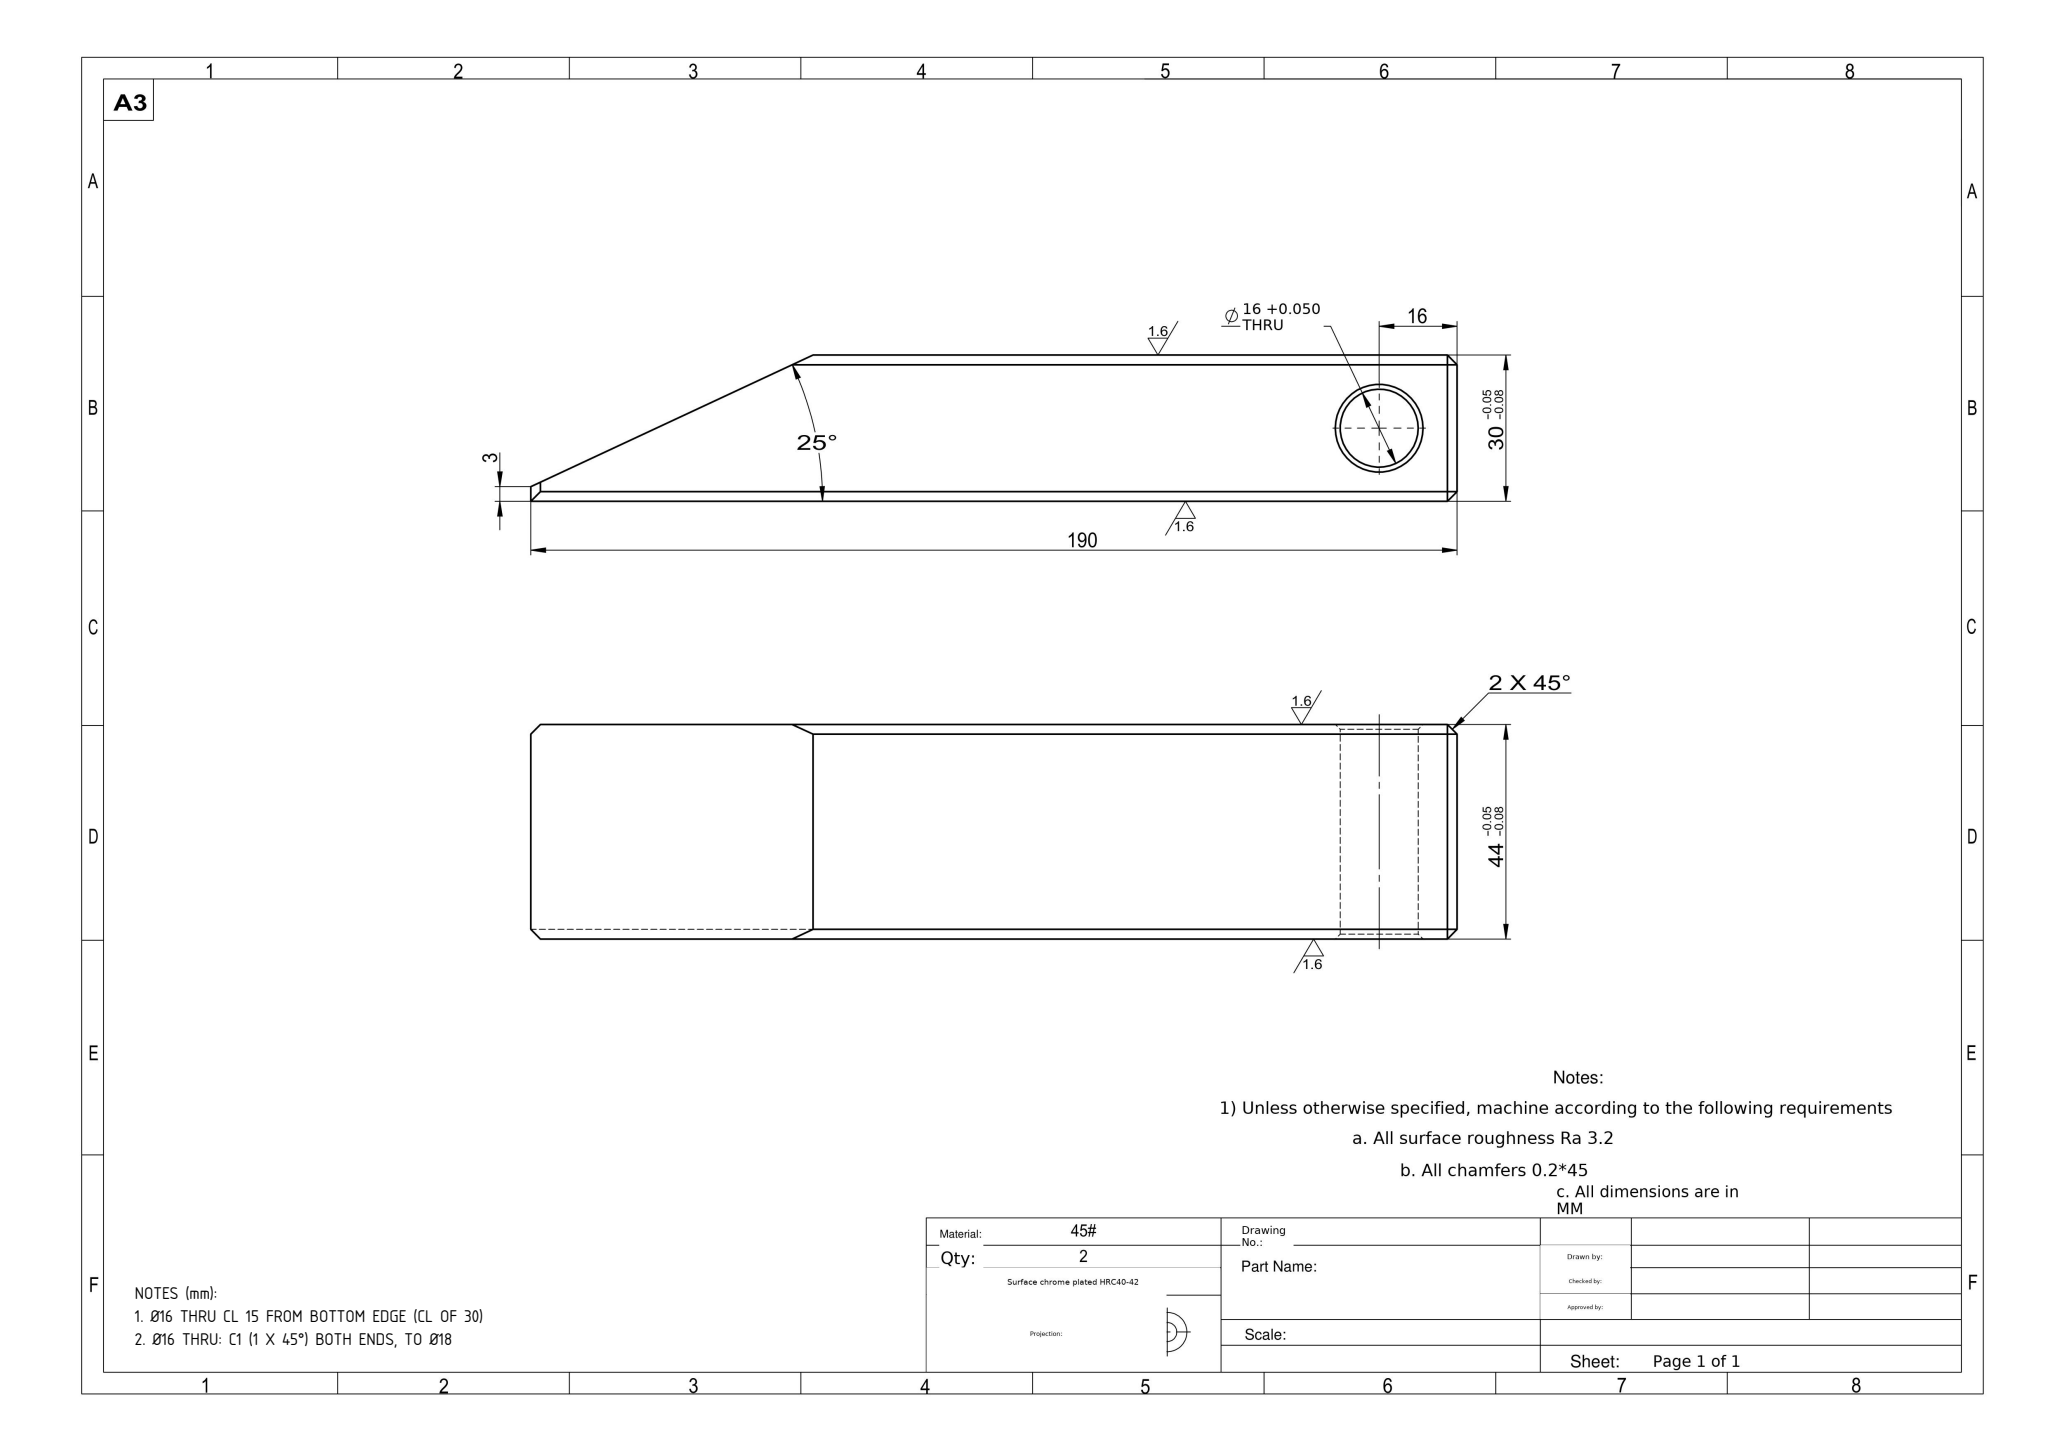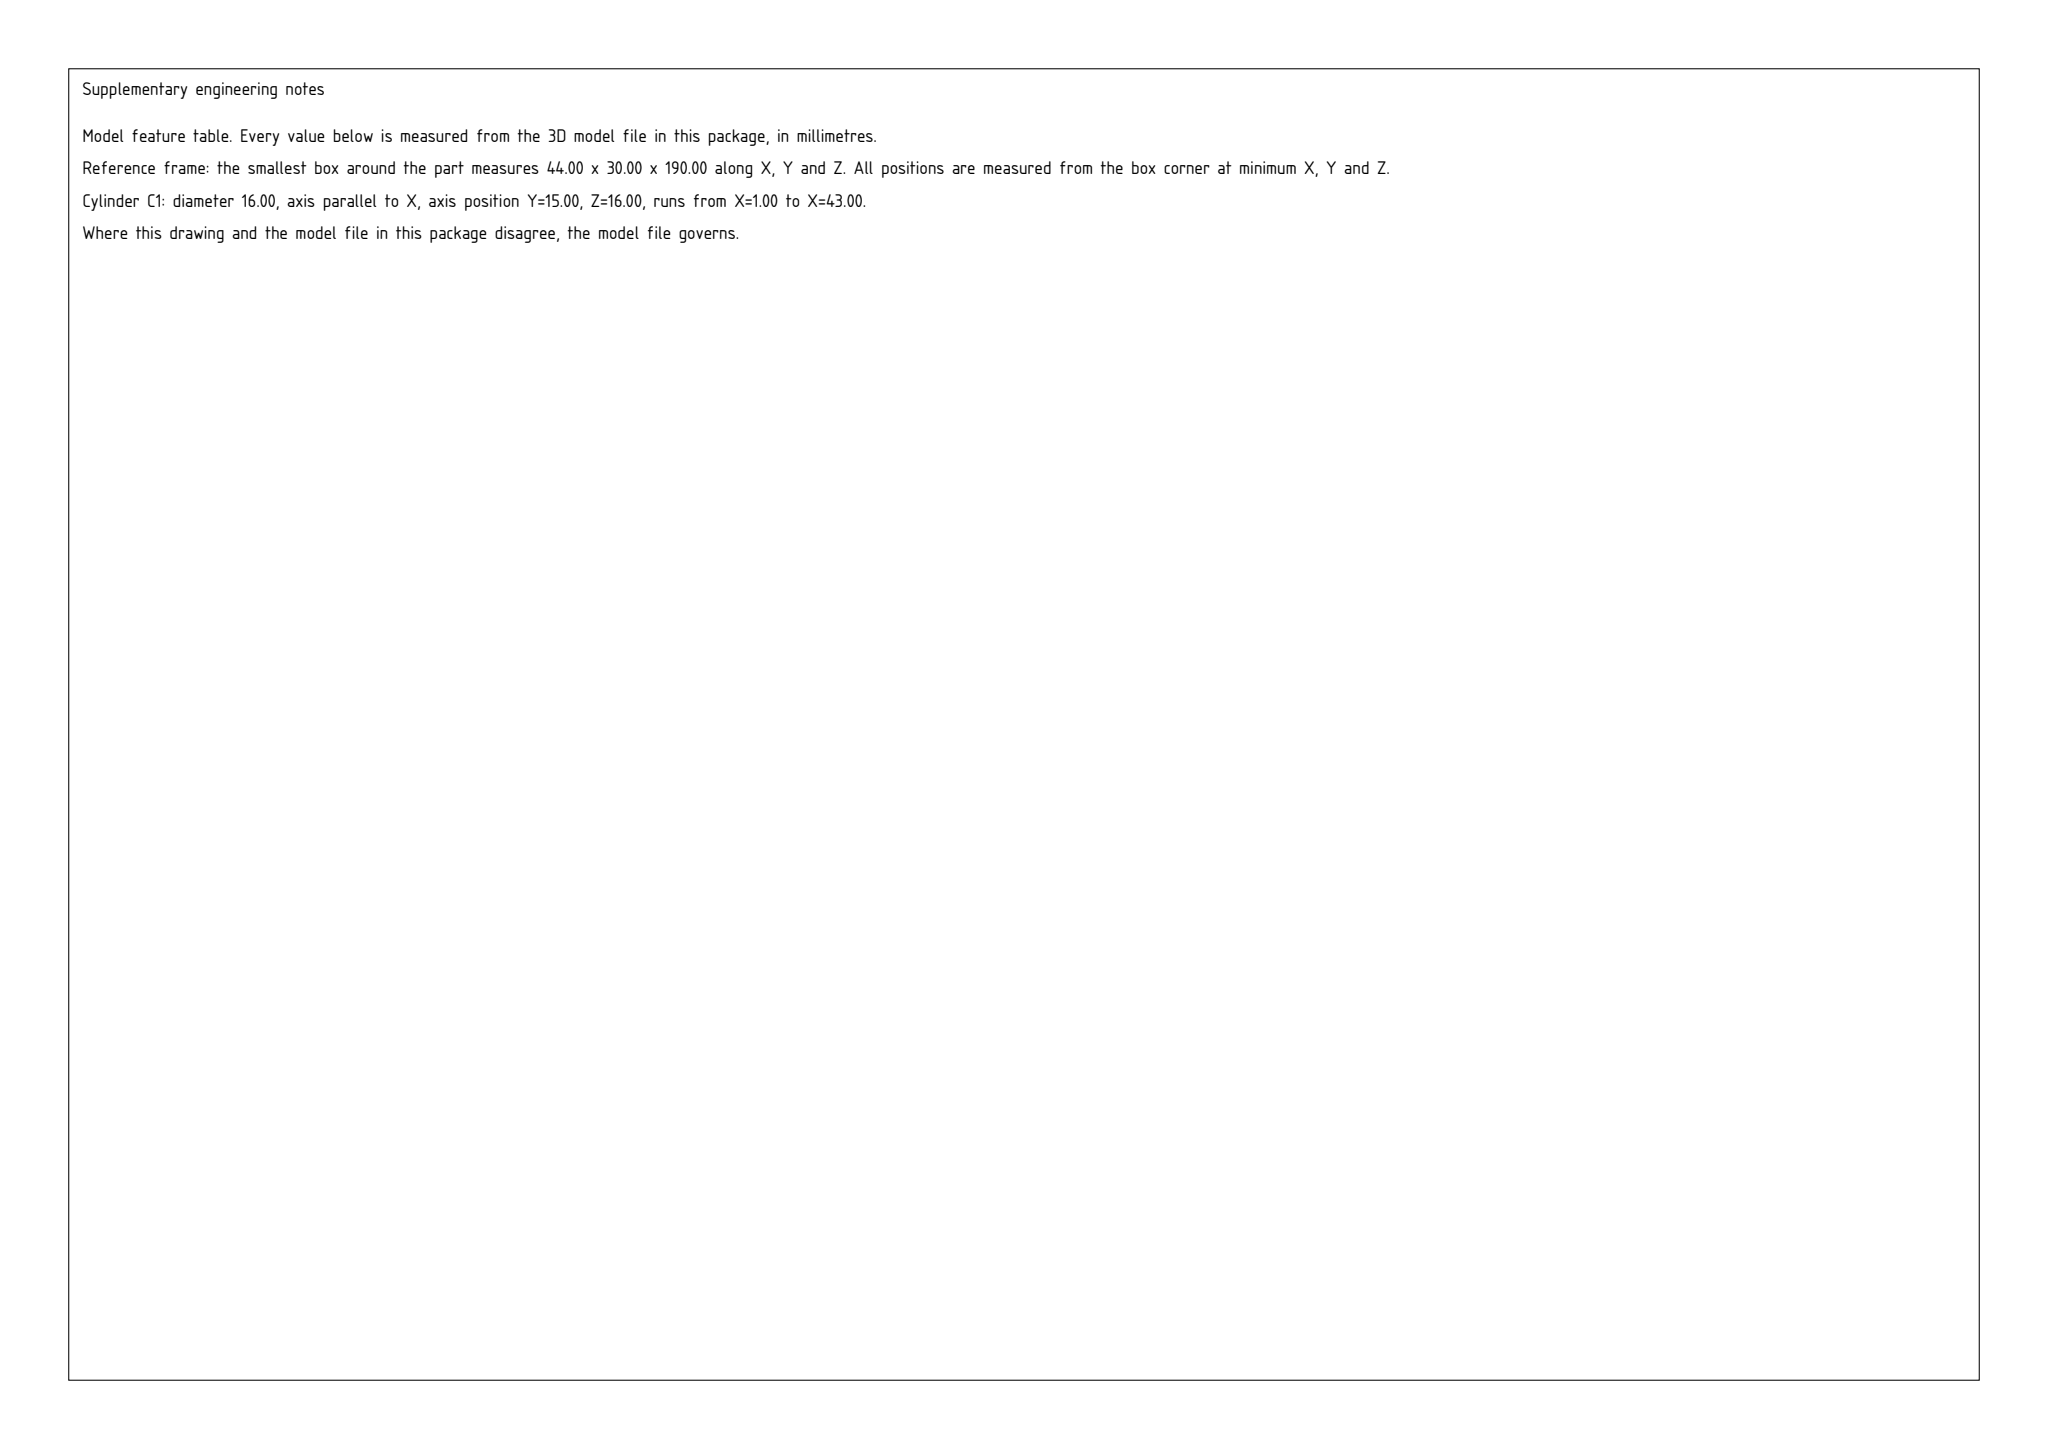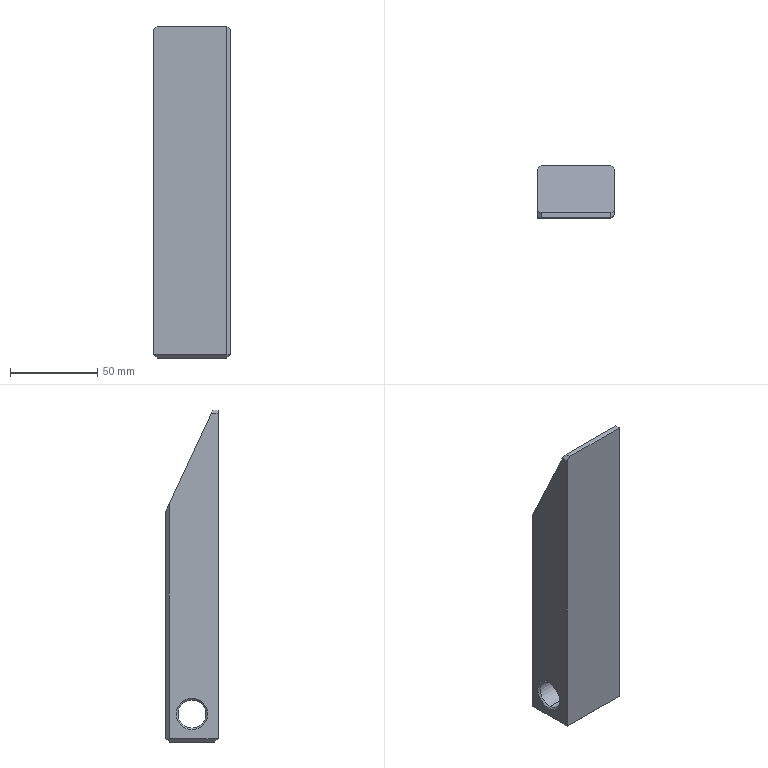Part | SolidWorks | mm | 1 solid | 25 faces | box 44 x 30 x 190 mm | volume 206305 mm3 | plane 19 | cone 4 | cylinder 2 | commonest cylinder face diameters 16 x2
Drawing notes:
Ø16 THRU CL 15 FROM BOTTOM EDGE (CL OF 30) | from the solid: cylinder dia 16, axis x, y=15 of 30 bbox height
Ø16 THRU: C1 (1 X 45°) BOTH ENDS, TO Ø18 | from the solid: cyl length 42 in 44 wide block; cones 90 incl, ref dia 18 at both ends
build123d program:
from build123d import *

# Parameters (mm, degrees)
BOSS_EXTRUDE1_DEPTH        = 22
F_16_0_16_DIAMETER_HOLE1_D = 16
CHAMFER1_SIZE              = 2
CHAMFER2_SIZE              = 1


with BuildPart() as part:
    # Sketch1 → Boss-Extrude1 (new, symmetric)
    with BuildSketch(Plane(origin=(0, 0, 0), x_dir=(0, 0, -1), z_dir=(1, 0, 0))):
        Polygon((-95, 0), (95, 0), (95, 30), (-37.098, 30), (-95, 3), align=None)
    extrude(amount=BOSS_EXTRUDE1_DEPTH, both=True)

    # 16.0 _16_ Diameter Hole1 (through all)
    with Locations(Plane(origin=(22, 0, 0), x_dir=(0, 0, -1), z_dir=(1, 0, 0))):
        with Locations((79, 15)):
            Hole(F_16_0_16_DIAMETER_HOLE1_D / 2)

    # Chamfer1
    chamfer1_edges = [part.edges().sort_by_distance(p)[0] for p in [
        (22, 15, -95),
        (22, 30, -28.951),
        (22, 1.5, 95),
        (-22, 30, -28.951),
        (-22, 15, -95),
        (-22, 1.5, 95),
        (22, 0, 0),
        (0, 30, -95),
        (0, 0, -95),
    ]]
    chamfer(chamfer1_edges, length=CHAMFER1_SIZE)

    # Chamfer2
    chamfer2_edges = [part.edges().sort_by_distance(p)[0] for p in [
        (22, 15, -87),
        (-22, 15, -87),
    ]]
    chamfer(chamfer2_edges, length=CHAMFER2_SIZE)


solid = part.part
STEP:
#1=CARTESIAN_POINT('',(-21.,15.,-87.));
#2=VERTEX_POINT('',#1);
#3=CARTESIAN_POINT('',(-21.,15.,-71.));
#4=VERTEX_POINT('',#3);
#5=CARTESIAN_POINT('',(-21.,15.,-79.));
#6=DIRECTION('',(-1.,0.,0.));
#7=DIRECTION('',(0.,0.,-1.));
#8=AXIS2_PLACEMENT_3D('',#5,#6,#7);
#9=CIRCLE('',#8,8.);
#10=EDGE_CURVE('',#2,#4,#9,.T.);
#11=ORIENTED_EDGE('',*,*,#10,.F.);
#12=CARTESIAN_POINT('',(-22.,15.,-88.));
#13=VERTEX_POINT('',#12);
#14=CARTESIAN_POINT('',(-22.,15.,-88.));
#15=DIRECTION('',(-0.7071,0.,-0.7071));
#16=VECTOR('',#15,1000.);
#17=LINE('',#14,#16);
#18=EDGE_CURVE('',#2,#13,#17,.T.);
#19=ORIENTED_EDGE('',*,*,#18,.T.);
#20=CARTESIAN_POINT('',(-22.,15.,-70.));
#21=VERTEX_POINT('',#20);
#22=CARTESIAN_POINT('',(-22.,15.,-79.));
#23=DIRECTION('',(1.,0.,0.));
#24=DIRECTION('',(0.,0.,-1.));
#25=AXIS2_PLACEMENT_3D('',#22,#23,#24);
#26=CIRCLE('',#25,9.);
#27=EDGE_CURVE('',#21,#13,#26,.T.);
#28=ORIENTED_EDGE('',*,*,#27,.F.);
#29=CARTESIAN_POINT('',(-22.,15.,-70.));
#30=DIRECTION('',(-0.7071,0.,0.7071));
#31=VECTOR('',#30,1000.);
#32=LINE('',#29,#31);
#33=EDGE_CURVE('',#4,#21,#32,.T.);
#34=ORIENTED_EDGE('',*,*,#33,.F.);
#35=EDGE_LOOP('',(#11,#19,#28,#34));
#36=FACE_OUTER_BOUND('',#35,.T.);
#37=CARTESIAN_POINT('',(-22.,15.,-79.));
#38=DIRECTION('',(-1.,0.,0.));
#39=DIRECTION('',(0.,0.,1.));
#40=AXIS2_PLACEMENT_3D('',#37,#38,#39);
#41=CONICAL_SURFACE('',#40,9.,0.7854);
#42=ADVANCED_FACE('',(#36),#41,.F.);
#43=CARTESIAN_POINT('',(21.,15.,-71.));
#44=VERTEX_POINT('',#43);
#45=CARTESIAN_POINT('',(21.,15.,-87.));
#46=VERTEX_POINT('',#45);
#47=CARTESIAN_POINT('',(21.,15.,-79.));
#48=DIRECTION('',(1.,0.,0.));
#49=DIRECTION('',(0.,0.,-1.));
#50=AXIS2_PLACEMENT_3D('',#47,#48,#49);
#51=CIRCLE('',#50,8.);
#52=EDGE_CURVE('',#44,#46,#51,.T.);
#53=ORIENTED_EDGE('',*,*,#52,.F.);
#54=CARTESIAN_POINT('',(22.,15.,-70.));
#55=VERTEX_POINT('',#54);
#56=CARTESIAN_POINT('',(21.,15.,-71.));
#57=DIRECTION('',(0.7071,0.,0.7071));
#58=VECTOR('',#57,1000.);
#59=LINE('',#56,#58);
#60=EDGE_CURVE('',#44,#55,#59,.T.);
#61=ORIENTED_EDGE('',*,*,#60,.T.);
#62=CARTESIAN_POINT('',(22.,15.,-88.));
#63=VERTEX_POINT('',#62);
#64=CARTESIAN_POINT('',(22.,15.,-79.));
#65=DIRECTION('',(-1.,0.,0.));
#66=DIRECTION('',(0.,0.,-1.));
#67=AXIS2_PLACEMENT_3D('',#64,#65,#66);
#68=CIRCLE('',#67,9.);
#69=EDGE_CURVE('',#63,#55,#68,.T.);
#70=ORIENTED_EDGE('',*,*,#69,.F.);
#71=CARTESIAN_POINT('',(21.,15.,-87.));
#72=DIRECTION('',(0.7071,0.,-0.7071));
#73=VECTOR('',#72,1000.);
#74=LINE('',#71,#73);
#75=EDGE_CURVE('',#46,#63,#74,.T.);
#76=ORIENTED_EDGE('',*,*,#75,.F.);
#77=EDGE_LOOP('',(#53,#61,#70,#76));
#78=FACE_OUTER_BOUND('',#77,.T.);
#79=CARTESIAN_POINT('',(21.,15.,-79.));
#80=DIRECTION('',(1.,0.,0.));
#81=DIRECTION('',(0.,0.,-1.));
#82=AXIS2_PLACEMENT_3D('',#79,#80,#81);
#83=CONICAL_SURFACE('',#82,8.,0.7854);
#84=ADVANCED_FACE('',(#78),#83,.F.);
#85=ORIENTED_EDGE('',*,*,#10,.T.);
#86=CARTESIAN_POINT('',(22.,15.,-71.));
#87=DIRECTION('',(1.,0.,0.));
#88=VECTOR('',#87,1000.);
#89=LINE('',#86,#88);
#90=EDGE_CURVE('',#4,#44,#89,.T.);
#91=ORIENTED_EDGE('',*,*,#90,.T.);
#92=ORIENTED_EDGE('',*,*,#52,.T.);
#93=CARTESIAN_POINT('',(22.,15.,-87.));
#94=DIRECTION('',(1.,0.,0.));
#95=VECTOR('',#94,1000.);
#96=LINE('',#93,#95);
#97=EDGE_CURVE('',#2,#46,#96,.T.);
#98=ORIENTED_EDGE('',*,*,#97,.F.);
#99=EDGE_LOOP('',(#85,#91,#92,#98));
#100=FACE_OUTER_BOUND('',#99,.T.);
#101=CARTESIAN_POINT('',(22.,15.,-79.));
#102=DIRECTION('',(1.,0.,0.));
#103=DIRECTION('',(0.,0.,-1.));
#104=AXIS2_PLACEMENT_3D('',#101,#102,#103);
#105=CYLINDRICAL_SURFACE('',#104,8.);
#106=ADVANCED_FACE('',(#100),#105,.F.);
#107=CARTESIAN_POINT('',(20.,3.,95.));
#108=VERTEX_POINT('',#107);
#109=CARTESIAN_POINT('',(-20.,3.,95.));
#110=VERTEX_POINT('',#109);
#111=CARTESIAN_POINT('',(22.,3.,95.));
#112=DIRECTION('',(-1.,0.,0.));
#113=VECTOR('',#112,1000.);
#114=LINE('',#111,#113);
#115=EDGE_CURVE('',#108,#110,#114,.T.);
#116=ORIENTED_EDGE('',*,*,#115,.T.);
#117=CARTESIAN_POINT('',(-20.,0.,95.));
#118=VERTEX_POINT('',#117);
#119=CARTESIAN_POINT('',(-20.,3.,95.));
#120=DIRECTION('',(0.,-1.,0.));
#121=VECTOR('',#120,1000.);
#122=LINE('',#119,#121);
#123=EDGE_CURVE('',#110,#118,#122,.T.);
#124=ORIENTED_EDGE('',*,*,#123,.T.);
#125=CARTESIAN_POINT('',(20.,0.,95.));
#126=VERTEX_POINT('',#125);
#127=CARTESIAN_POINT('',(22.,0.,95.));
#128=DIRECTION('',(-1.,0.,0.));
#129=VECTOR('',#128,1000.);
#130=LINE('',#127,#129);
#131=EDGE_CURVE('',#126,#118,#130,.T.);
#132=ORIENTED_EDGE('',*,*,#131,.F.);
#133=CARTESIAN_POINT('',(20.,3.,95.));
#134=DIRECTION('',(0.,1.,0.));
#135=VECTOR('',#134,1000.);
#136=LINE('',#133,#135);
#137=EDGE_CURVE('',#126,#108,#136,.T.);
#138=ORIENTED_EDGE('',*,*,#137,.T.);
#139=EDGE_LOOP('',(#116,#124,#132,#138));
#140=FACE_OUTER_BOUND('',#139,.T.);
#141=CARTESIAN_POINT('',(22.,3.,95.));
#142=DIRECTION('',(0.,0.,-1.));
#143=DIRECTION('',(-1.,0.,0.));
#144=AXIS2_PLACEMENT_3D('',#141,#142,#143);
#145=PLANE('',#144);
#146=ADVANCED_FACE('',(#140),#145,.F.);
#147=ORIENTED_EDGE('',*,*,#131,.T.);
#148=CARTESIAN_POINT('',(-22.,0.,93.));
#149=VERTEX_POINT('',#148);
#150=CARTESIAN_POINT('',(-20.,0.,95.));
#151=DIRECTION('',(-0.7071,0.,-0.7071));
#152=VECTOR('',#151,1000.);
#153=LINE('',#150,#152);
#154=EDGE_CURVE('',#118,#149,#153,.T.);
#155=ORIENTED_EDGE('',*,*,#154,.T.);
#156=CARTESIAN_POINT('',(-22.,0.,-93.));
#157=VERTEX_POINT('',#156);
#158=CARTESIAN_POINT('',(-22.,0.,95.));
#159=DIRECTION('',(0.,0.,-1.));
#160=VECTOR('',#159,1000.);
#161=LINE('',#158,#160);
#162=EDGE_CURVE('',#149,#157,#161,.T.);
#163=ORIENTED_EDGE('',*,*,#162,.T.);
#164=CARTESIAN_POINT('',(20.,0.,-93.));
#165=VERTEX_POINT('',#164);
#166=CARTESIAN_POINT('',(22.,0.,-93.));
#167=DIRECTION('',(1.,0.,0.));
#168=VECTOR('',#167,1000.);
#169=LINE('',#166,#168);
#170=EDGE_CURVE('',#157,#165,#169,.T.);
#171=ORIENTED_EDGE('',*,*,#170,.T.);
#172=CARTESIAN_POINT('',(20.,0.,95.));
#173=DIRECTION('',(0.,0.,1.));
#174=VECTOR('',#173,1000.);
#175=LINE('',#172,#174);
#176=EDGE_CURVE('',#165,#126,#175,.T.);
#177=ORIENTED_EDGE('',*,*,#176,.T.);
#178=EDGE_LOOP('',(#147,#155,#163,#171,#177));
#179=FACE_OUTER_BOUND('',#178,.T.);
#180=CARTESIAN_POINT('',(22.,0.,95.));
#181=DIRECTION('',(0.,1.,0.));
#182=DIRECTION('',(0.,0.,1.));
#183=AXIS2_PLACEMENT_3D('',#180,#181,#182);
#184=PLANE('',#183);
#185=ADVANCED_FACE('',(#179),#184,.F.);
#186=CARTESIAN_POINT('',(20.,28.,-95.));
#187=VERTEX_POINT('',#186);
#188=CARTESIAN_POINT('',(20.,2.,-95.));
#189=VERTEX_POINT('',#188);
#190=CARTESIAN_POINT('',(20.,0.,-95.));
#191=DIRECTION('',(0.,-1.,0.));
#192=VECTOR('',#191,1000.);
#193=LINE('',#190,#192);
#194=EDGE_CURVE('',#187,#189,#193,.T.);
#195=ORIENTED_EDGE('',*,*,#194,.T.);
#196=CARTESIAN_POINT('',(-20.,2.,-95.));
#197=VERTEX_POINT('',#196);
#198=CARTESIAN_POINT('',(22.,2.,-95.));
#199=DIRECTION('',(-1.,0.,0.));
#200=VECTOR('',#199,1000.);
#201=LINE('',#198,#200);
#202=EDGE_CURVE('',#189,#197,#201,.T.);
#203=ORIENTED_EDGE('',*,*,#202,.T.);
#204=CARTESIAN_POINT('',(-20.,28.,-95.));
#205=VERTEX_POINT('',#204);
#206=CARTESIAN_POINT('',(-20.,0.,-95.));
#207=DIRECTION('',(0.,1.,0.));
#208=VECTOR('',#207,1000.);
#209=LINE('',#206,#208);
#210=EDGE_CURVE('',#197,#205,#209,.T.);
#211=ORIENTED_EDGE('',*,*,#210,.T.);
#212=CARTESIAN_POINT('',(22.,28.,-95.));
#213=DIRECTION('',(1.,0.,0.));
#214=VECTOR('',#213,1000.);
#215=LINE('',#212,#214);
#216=EDGE_CURVE('',#205,#187,#215,.T.);
#217=ORIENTED_EDGE('',*,*,#216,.T.);
#218=EDGE_LOOP('',(#195,#203,#211,#217));
#219=FACE_OUTER_BOUND('',#218,.T.);
#220=CARTESIAN_POINT('',(22.,0.,-95.));
#221=DIRECTION('',(0.,0.,1.));
#222=DIRECTION('',(1.,0.,0.));
#223=AXIS2_PLACEMENT_3D('',#220,#221,#222);
#224=PLANE('',#223);
#225=ADVANCED_FACE('',(#219),#224,.F.);
#226=CARTESIAN_POINT('',(20.,30.,-93.));
#227=VERTEX_POINT('',#226);
#228=CARTESIAN_POINT('',(-20.,30.,-93.));
#229=VERTEX_POINT('',#228);
#230=CARTESIAN_POINT('',(22.,30.,-93.));
#231=DIRECTION('',(-1.,0.,0.));
#232=VECTOR('',#231,1000.);
#233=LINE('',#230,#232);
#234=EDGE_CURVE('',#227,#229,#233,.T.);
#235=ORIENTED_EDGE('',*,*,#234,.T.);
#236=CARTESIAN_POINT('',(-20.,30.,37.098));
#237=VERTEX_POINT('',#236);
#238=CARTESIAN_POINT('',(-20.,30.,-95.));
#239=DIRECTION('',(0.,-0.,1.));
#240=VECTOR('',#239,1000.);
#241=LINE('',#238,#240);
#242=EDGE_CURVE('',#229,#237,#241,.T.);
#243=ORIENTED_EDGE('',*,*,#242,.T.);
#244=CARTESIAN_POINT('',(20.,30.,37.098));
#245=VERTEX_POINT('',#244);
#246=CARTESIAN_POINT('',(22.,30.,37.098));
#247=DIRECTION('',(-1.,0.,0.));
#248=VECTOR('',#247,1000.);
#249=LINE('',#246,#248);
#250=EDGE_CURVE('',#245,#237,#249,.T.);
#251=ORIENTED_EDGE('',*,*,#250,.F.);
#252=CARTESIAN_POINT('',(20.,30.,-95.));
#253=DIRECTION('',(0.,0.,-1.));
#254=VECTOR('',#253,1000.);
#255=LINE('',#252,#254);
#256=EDGE_CURVE('',#245,#227,#255,.T.);
#257=ORIENTED_EDGE('',*,*,#256,.T.);
#258=EDGE_LOOP('',(#235,#243,#251,#257));
#259=FACE_OUTER_BOUND('',#258,.T.);
#260=CARTESIAN_POINT('',(22.,30.,-95.));
#261=DIRECTION('',(0.,-1.,-0.));
#262=DIRECTION('',(0.,0.,-1.));
#263=AXIS2_PLACEMENT_3D('',#260,#261,#262);
#264=PLANE('',#263);
#265=ADVANCED_FACE('',(#259),#264,.F.);
#266=CARTESIAN_POINT('',(-22.,28.,41.387));
#267=VERTEX_POINT('',#266);
#268=CARTESIAN_POINT('',(-22.,3.933,93.));
#269=VERTEX_POINT('',#268);
#270=CARTESIAN_POINT('',(-22.,30.,37.098));
#271=DIRECTION('',(0.,-0.4226,0.9063));
#272=VECTOR('',#271,1000.);
#273=LINE('',#270,#272);
#274=EDGE_CURVE('',#267,#269,#273,.T.);
#275=ORIENTED_EDGE('',*,*,#274,.T.);
#276=CARTESIAN_POINT('',(-20.,3.,95.));
#277=DIRECTION('',(0.6715,-0.3131,0.6715));
#278=VECTOR('',#277,1000.);
#279=LINE('',#276,#278);
#280=EDGE_CURVE('',#269,#110,#279,.T.);
#281=ORIENTED_EDGE('',*,*,#280,.T.);
#282=ORIENTED_EDGE('',*,*,#115,.F.);
#283=CARTESIAN_POINT('',(22.,3.933,93.));
#284=VERTEX_POINT('',#283);
#285=CARTESIAN_POINT('',(21.173,3.547,93.827));
#286=DIRECTION('',(0.6715,0.3131,-0.6715));
#287=VECTOR('',#286,1000.);
#288=LINE('',#285,#287);
#289=EDGE_CURVE('',#108,#284,#288,.T.);
#290=ORIENTED_EDGE('',*,*,#289,.T.);
#291=CARTESIAN_POINT('',(22.,28.,41.387));
#292=VERTEX_POINT('',#291);
#293=CARTESIAN_POINT('',(22.,30.,37.098));
#294=DIRECTION('',(0.,-0.4226,0.9063));
#295=VECTOR('',#294,1000.);
#296=LINE('',#293,#295);
#297=EDGE_CURVE('',#292,#284,#296,.T.);
#298=ORIENTED_EDGE('',*,*,#297,.F.);
#299=CARTESIAN_POINT('',(8.55,41.45,12.544));
#300=DIRECTION('',(-0.3893,0.3893,-0.8348));
#301=VECTOR('',#300,1000.);
#302=LINE('',#299,#301);
#303=EDGE_CURVE('',#292,#245,#302,.T.);
#304=ORIENTED_EDGE('',*,*,#303,.T.);
#305=ORIENTED_EDGE('',*,*,#250,.T.);
#306=CARTESIAN_POINT('',(22.929,72.929,-54.964));
#307=DIRECTION('',(-0.3893,-0.3893,0.8348));
#308=VECTOR('',#307,1000.);
#309=LINE('',#306,#308);
#310=EDGE_CURVE('',#237,#267,#309,.T.);
#311=ORIENTED_EDGE('',*,*,#310,.T.);
#312=EDGE_LOOP('',(#275,#281,#282,#290,#298,#304,#305,#311));
#313=FACE_OUTER_BOUND('',#312,.T.);
#314=CARTESIAN_POINT('',(22.,30.,37.098));
#315=DIRECTION('',(0.,-0.9063,-0.4226));
#316=DIRECTION('',(0.,0.4226,-0.9063));
#317=AXIS2_PLACEMENT_3D('',#314,#315,#316);
#318=PLANE('',#317);
#319=ADVANCED_FACE('',(#313),#318,.F.);
#320=ORIENTED_EDGE('',*,*,#69,.T.);
#321=CARTESIAN_POINT('',(22.,15.,-79.));
#322=DIRECTION('',(-1.,0.,0.));
#323=DIRECTION('',(0.,0.,-1.));
#324=AXIS2_PLACEMENT_3D('',#321,#322,#323);
#325=CIRCLE('',#324,9.);
#326=EDGE_CURVE('',#55,#63,#325,.T.);
#327=ORIENTED_EDGE('',*,*,#326,.T.);
#328=EDGE_LOOP('',(#320,#327));
#329=FACE_BOUND('',#328,.T.);
#330=CARTESIAN_POINT('',(22.,2.,-93.));
#331=VERTEX_POINT('',#330);
#332=CARTESIAN_POINT('',(22.,28.,-93.));
#333=VERTEX_POINT('',#332);
#334=CARTESIAN_POINT('',(22.,30.,-93.));
#335=DIRECTION('',(0.,1.,0.));
#336=VECTOR('',#335,1000.);
#337=LINE('',#334,#336);
#338=EDGE_CURVE('',#331,#333,#337,.T.);
#339=ORIENTED_EDGE('',*,*,#338,.T.);
#340=CARTESIAN_POINT('',(22.,28.,37.098));
#341=DIRECTION('',(0.,-0.,1.));
#342=VECTOR('',#341,1000.);
#343=LINE('',#340,#342);
#344=EDGE_CURVE('',#333,#292,#343,.T.);
#345=ORIENTED_EDGE('',*,*,#344,.T.);
#346=ORIENTED_EDGE('',*,*,#297,.T.);
#347=CARTESIAN_POINT('',(22.,2.,93.));
#348=VERTEX_POINT('',#347);
#349=CARTESIAN_POINT('',(22.,0.,93.));
#350=DIRECTION('',(0.,-1.,0.));
#351=VECTOR('',#350,1000.);
#352=LINE('',#349,#351);
#353=EDGE_CURVE('',#284,#348,#352,.T.);
#354=ORIENTED_EDGE('',*,*,#353,.T.);
#355=CARTESIAN_POINT('',(22.,2.,-95.));
#356=DIRECTION('',(0.,0.,-1.));
#357=VECTOR('',#356,1000.);
#358=LINE('',#355,#357);
#359=EDGE_CURVE('',#348,#331,#358,.T.);
#360=ORIENTED_EDGE('',*,*,#359,.T.);
#361=EDGE_LOOP('',(#339,#345,#346,#354,#360));
#362=FACE_OUTER_BOUND('',#361,.T.);
#363=CARTESIAN_POINT('',(22.,0.,0.));
#364=DIRECTION('',(1.,0.,0.));
#365=DIRECTION('',(0.,0.,-1.));
#366=AXIS2_PLACEMENT_3D('',#363,#364,#365);
#367=PLANE('',#366);
#368=ADVANCED_FACE('',(#329,#362),#367,.T.);
#369=ORIENTED_EDGE('',*,*,#27,.T.);
#370=CARTESIAN_POINT('',(-22.,15.,-79.));
#371=DIRECTION('',(1.,0.,0.));
#372=DIRECTION('',(0.,0.,-1.));
#373=AXIS2_PLACEMENT_3D('',#370,#371,#372);
#374=CIRCLE('',#373,9.);
#375=EDGE_CURVE('',#13,#21,#374,.T.);
#376=ORIENTED_EDGE('',*,*,#375,.T.);
#377=EDGE_LOOP('',(#369,#376));
#378=FACE_BOUND('',#377,.T.);
#379=ORIENTED_EDGE('',*,*,#162,.F.);
#380=CARTESIAN_POINT('',(-22.,0.,93.));
#381=DIRECTION('',(0.,1.,0.));
#382=VECTOR('',#381,1000.);
#383=LINE('',#380,#382);
#384=EDGE_CURVE('',#149,#269,#383,.T.);
#385=ORIENTED_EDGE('',*,*,#384,.T.);
#386=ORIENTED_EDGE('',*,*,#274,.F.);
#387=CARTESIAN_POINT('',(-22.,28.,-93.));
#388=VERTEX_POINT('',#387);
#389=CARTESIAN_POINT('',(-22.,28.,0.));
#390=DIRECTION('',(0.,0.,-1.));
#391=VECTOR('',#390,1000.);
#392=LINE('',#389,#391);
#393=EDGE_CURVE('',#267,#388,#392,.T.);
#394=ORIENTED_EDGE('',*,*,#393,.T.);
#395=CARTESIAN_POINT('',(-22.,0.,-93.));
#396=DIRECTION('',(0.,-1.,0.));
#397=VECTOR('',#396,1000.);
#398=LINE('',#395,#397);
#399=EDGE_CURVE('',#388,#157,#398,.T.);
#400=ORIENTED_EDGE('',*,*,#399,.T.);
#401=EDGE_LOOP('',(#379,#385,#386,#394,#400));
#402=FACE_OUTER_BOUND('',#401,.T.);
#403=CARTESIAN_POINT('',(-22.,0.,0.));
#404=DIRECTION('',(1.,0.,0.));
#405=DIRECTION('',(0.,0.,-1.));
#406=AXIS2_PLACEMENT_3D('',#403,#404,#405);
#407=PLANE('',#406);
#408=ADVANCED_FACE('',(#378,#402),#407,.F.);
#409=ORIENTED_EDGE('',*,*,#90,.F.);
#410=CARTESIAN_POINT('',(-21.,15.,-79.));
#411=DIRECTION('',(-1.,0.,0.));
#412=DIRECTION('',(0.,0.,-1.));
#413=AXIS2_PLACEMENT_3D('',#410,#411,#412);
#414=CIRCLE('',#413,8.);
#415=EDGE_CURVE('',#4,#2,#414,.T.);
#416=ORIENTED_EDGE('',*,*,#415,.T.);
#417=ORIENTED_EDGE('',*,*,#97,.T.);
#418=CARTESIAN_POINT('',(21.,15.,-79.));
#419=DIRECTION('',(1.,0.,0.));
#420=DIRECTION('',(0.,0.,-1.));
#421=AXIS2_PLACEMENT_3D('',#418,#419,#420);
#422=CIRCLE('',#421,8.);
#423=EDGE_CURVE('',#46,#44,#422,.T.);
#424=ORIENTED_EDGE('',*,*,#423,.T.);
#425=EDGE_LOOP('',(#409,#416,#417,#424));
#426=FACE_OUTER_BOUND('',#425,.T.);
#427=CARTESIAN_POINT('',(22.,15.,-79.));
#428=DIRECTION('',(1.,0.,0.));
#429=DIRECTION('',(0.,0.,-1.));
#430=AXIS2_PLACEMENT_3D('',#427,#428,#429);
#431=CYLINDRICAL_SURFACE('',#430,8.);
#432=ADVANCED_FACE('',(#426),#431,.F.);
#433=ORIENTED_EDGE('',*,*,#280,.F.);
#434=ORIENTED_EDGE('',*,*,#384,.F.);
#435=ORIENTED_EDGE('',*,*,#154,.F.);
#436=ORIENTED_EDGE('',*,*,#123,.F.);
#437=EDGE_LOOP('',(#433,#434,#435,#436));
#438=FACE_OUTER_BOUND('',#437,.T.);
#439=CARTESIAN_POINT('',(-20.,3.,95.));
#440=DIRECTION('',(0.7071,0.,-0.7071));
#441=DIRECTION('',(0.,-1.,0.));
#442=AXIS2_PLACEMENT_3D('',#439,#440,#441);
#443=PLANE('',#442);
#444=ADVANCED_FACE('',(#438),#443,.F.);
#445=ORIENTED_EDGE('',*,*,#303,.F.);
#446=ORIENTED_EDGE('',*,*,#344,.F.);
#447=CARTESIAN_POINT('',(21.,29.,-93.));
#448=DIRECTION('',(0.7071,-0.7071,-0.));
#449=VECTOR('',#448,1000.);
#450=LINE('',#447,#449);
#451=EDGE_CURVE('',#227,#333,#450,.T.);
#452=ORIENTED_EDGE('',*,*,#451,.F.);
#453=ORIENTED_EDGE('',*,*,#256,.F.);
#454=EDGE_LOOP('',(#445,#446,#452,#453));
#455=FACE_OUTER_BOUND('',#454,.T.);
#456=CARTESIAN_POINT('',(22.,28.,0.));
#457=DIRECTION('',(0.7071,0.7071,0.));
#458=DIRECTION('',(0.,0.,-1.));
#459=AXIS2_PLACEMENT_3D('',#456,#457,#458);
#460=PLANE('',#459);
#461=ADVANCED_FACE('',(#455),#460,.T.);
#462=ORIENTED_EDGE('',*,*,#289,.F.);
#463=ORIENTED_EDGE('',*,*,#137,.F.);
#464=CARTESIAN_POINT('',(21.333,1.333,93.667));
#465=DIRECTION('',(-0.5774,-0.5774,0.5774));
#466=VECTOR('',#465,1000.);
#467=LINE('',#464,#466);
#468=EDGE_CURVE('',#348,#126,#467,.T.);
#469=ORIENTED_EDGE('',*,*,#468,.F.);
#470=ORIENTED_EDGE('',*,*,#353,.F.);
#471=EDGE_LOOP('',(#462,#463,#469,#470));
#472=FACE_OUTER_BOUND('',#471,.T.);
#473=CARTESIAN_POINT('',(22.,0.,93.));
#474=DIRECTION('',(0.7071,0.,0.7071));
#475=DIRECTION('',(0.,1.,0.));
#476=AXIS2_PLACEMENT_3D('',#473,#474,#475);
#477=PLANE('',#476);
#478=ADVANCED_FACE('',(#472),#477,.T.);
#479=CARTESIAN_POINT('',(20.,28.,-95.));
#480=DIRECTION('',(0.7071,0.,0.7071));
#481=VECTOR('',#480,1000.);
#482=LINE('',#479,#481);
#483=EDGE_CURVE('',#187,#333,#482,.T.);
#484=ORIENTED_EDGE('',*,*,#483,.F.);
#485=CARTESIAN_POINT('',(20.,28.,-95.));
#486=DIRECTION('',(0.,-0.7071,-0.7071));
#487=VECTOR('',#486,1000.);
#488=LINE('',#485,#487);
#489=EDGE_CURVE('',#227,#187,#488,.T.);
#490=ORIENTED_EDGE('',*,*,#489,.F.);
#491=ORIENTED_EDGE('',*,*,#451,.T.);
#492=EDGE_LOOP('',(#484,#490,#491));
#493=FACE_OUTER_BOUND('',#492,.T.);
#494=CARTESIAN_POINT('',(20.,28.,-95.));
#495=DIRECTION('',(0.5774,0.5774,-0.5774));
#496=DIRECTION('',(0.,0.7071,0.7071));
#497=AXIS2_PLACEMENT_3D('',#494,#495,#496);
#498=PLANE('',#497);
#499=ADVANCED_FACE('',(#493),#498,.T.);
#500=ORIENTED_EDGE('',*,*,#489,.T.);
#501=ORIENTED_EDGE('',*,*,#216,.F.);
#502=CARTESIAN_POINT('',(-20.,28.,-95.));
#503=DIRECTION('',(-0.,-0.7071,-0.7071));
#504=VECTOR('',#503,1000.);
#505=LINE('',#502,#504);
#506=EDGE_CURVE('',#229,#205,#505,.T.);
#507=ORIENTED_EDGE('',*,*,#506,.F.);
#508=ORIENTED_EDGE('',*,*,#234,.F.);
#509=EDGE_LOOP('',(#500,#501,#507,#508));
#510=FACE_OUTER_BOUND('',#509,.T.);
#511=CARTESIAN_POINT('',(22.,30.,-93.));
#512=DIRECTION('',(0.,-0.7071,0.7071));
#513=DIRECTION('',(-1.,0.,0.));
#514=AXIS2_PLACEMENT_3D('',#511,#512,#513);
#515=PLANE('',#514);
#516=ADVANCED_FACE('',(#510),#515,.F.);
#517=ORIENTED_EDGE('',*,*,#310,.F.);
#518=ORIENTED_EDGE('',*,*,#242,.F.);
#519=CARTESIAN_POINT('',(-21.,29.,-93.));
#520=DIRECTION('',(0.7071,0.7071,-0.));
#521=VECTOR('',#520,1000.);
#522=LINE('',#519,#521);
#523=EDGE_CURVE('',#388,#229,#522,.T.);
#524=ORIENTED_EDGE('',*,*,#523,.F.);
#525=ORIENTED_EDGE('',*,*,#393,.F.);
#526=EDGE_LOOP('',(#517,#518,#524,#525));
#527=FACE_OUTER_BOUND('',#526,.T.);
#528=CARTESIAN_POINT('',(-20.,30.,-95.));
#529=DIRECTION('',(0.7071,-0.7071,-0.));
#530=DIRECTION('',(0.,-0.,1.));
#531=AXIS2_PLACEMENT_3D('',#528,#529,#530);
#532=PLANE('',#531);
#533=ADVANCED_FACE('',(#527),#532,.F.);
#534=ORIENTED_EDGE('',*,*,#468,.T.);
#535=ORIENTED_EDGE('',*,*,#176,.F.);
#536=CARTESIAN_POINT('',(20.,0.,-93.));
#537=DIRECTION('',(-0.7071,-0.7071,0.));
#538=VECTOR('',#537,1000.);
#539=LINE('',#536,#538);
#540=EDGE_CURVE('',#331,#165,#539,.T.);
#541=ORIENTED_EDGE('',*,*,#540,.F.);
#542=ORIENTED_EDGE('',*,*,#359,.F.);
#543=EDGE_LOOP('',(#534,#535,#541,#542));
#544=FACE_OUTER_BOUND('',#543,.T.);
#545=CARTESIAN_POINT('',(22.,2.,0.));
#546=DIRECTION('',(0.7071,-0.7071,0.));
#547=DIRECTION('',(0.,0.,1.));
#548=AXIS2_PLACEMENT_3D('',#545,#546,#547);
#549=PLANE('',#548);
#550=ADVANCED_FACE('',(#544),#549,.T.);
#551=ORIENTED_EDGE('',*,*,#483,.T.);
#552=ORIENTED_EDGE('',*,*,#338,.F.);
#553=CARTESIAN_POINT('',(21.,2.,-94.));
#554=DIRECTION('',(0.7071,-0.,0.7071));
#555=VECTOR('',#554,1000.);
#556=LINE('',#553,#555);
#557=EDGE_CURVE('',#189,#331,#556,.T.);
#558=ORIENTED_EDGE('',*,*,#557,.F.);
#559=ORIENTED_EDGE('',*,*,#194,.F.);
#560=EDGE_LOOP('',(#551,#552,#558,#559));
#561=FACE_OUTER_BOUND('',#560,.T.);
#562=CARTESIAN_POINT('',(22.,0.,-93.));
#563=DIRECTION('',(0.7071,0.,-0.7071));
#564=DIRECTION('',(0.,-1.,0.));
#565=AXIS2_PLACEMENT_3D('',#562,#563,#564);
#566=PLANE('',#565);
#567=ADVANCED_FACE('',(#561),#566,.T.);
#568=ORIENTED_EDGE('',*,*,#523,.T.);
#569=ORIENTED_EDGE('',*,*,#506,.T.);
#570=CARTESIAN_POINT('',(-20.,28.,-95.));
#571=DIRECTION('',(0.7071,0.,-0.7071));
#572=VECTOR('',#571,1000.);
#573=LINE('',#570,#572);
#574=EDGE_CURVE('',#388,#205,#573,.T.);
#575=ORIENTED_EDGE('',*,*,#574,.F.);
#576=EDGE_LOOP('',(#568,#569,#575));
#577=FACE_OUTER_BOUND('',#576,.T.);
#578=CARTESIAN_POINT('',(-20.,28.,-95.));
#579=DIRECTION('',(-0.5774,0.5774,-0.5774));
#580=DIRECTION('',(-0.7071,0.,0.7071));
#581=AXIS2_PLACEMENT_3D('',#578,#579,#580);
#582=PLANE('',#581);
#583=ADVANCED_FACE('',(#577),#582,.T.);
#584=ORIENTED_EDGE('',*,*,#557,.T.);
#585=ORIENTED_EDGE('',*,*,#540,.T.);
#586=CARTESIAN_POINT('',(20.,0.,-93.));
#587=DIRECTION('',(-0.,-0.7071,0.7071));
#588=VECTOR('',#587,1000.);
#589=LINE('',#586,#588);
#590=EDGE_CURVE('',#189,#165,#589,.T.);
#591=ORIENTED_EDGE('',*,*,#590,.F.);
#592=EDGE_LOOP('',(#584,#585,#591));
#593=FACE_OUTER_BOUND('',#592,.T.);
#594=CARTESIAN_POINT('',(20.,0.,-93.));
#595=DIRECTION('',(0.5774,-0.5774,-0.5774));
#596=DIRECTION('',(0.,0.7071,-0.7071));
#597=AXIS2_PLACEMENT_3D('',#594,#595,#596);
#598=PLANE('',#597);
#599=ADVANCED_FACE('',(#593),#598,.T.);
#600=ORIENTED_EDGE('',*,*,#574,.T.);
#601=ORIENTED_EDGE('',*,*,#210,.F.);
#602=CARTESIAN_POINT('',(-20.667,1.333,-94.333));
#603=DIRECTION('',(0.5774,0.5774,-0.5774));
#604=VECTOR('',#603,1000.);
#605=LINE('',#602,#604);
#606=EDGE_CURVE('',#157,#197,#605,.T.);
#607=ORIENTED_EDGE('',*,*,#606,.F.);
#608=ORIENTED_EDGE('',*,*,#399,.F.);
#609=EDGE_LOOP('',(#600,#601,#607,#608));
#610=FACE_OUTER_BOUND('',#609,.T.);
#611=CARTESIAN_POINT('',(-20.,0.,-95.));
#612=DIRECTION('',(0.7071,0.,0.7071));
#613=DIRECTION('',(0.,1.,0.));
#614=AXIS2_PLACEMENT_3D('',#611,#612,#613);
#615=PLANE('',#614);
#616=ADVANCED_FACE('',(#610),#615,.F.);
#617=ORIENTED_EDGE('',*,*,#590,.T.);
#618=ORIENTED_EDGE('',*,*,#170,.F.);
#619=ORIENTED_EDGE('',*,*,#606,.T.);
#620=ORIENTED_EDGE('',*,*,#202,.F.);
#621=EDGE_LOOP('',(#617,#618,#619,#620));
#622=FACE_OUTER_BOUND('',#621,.T.);
#623=CARTESIAN_POINT('',(22.,2.,-95.));
#624=DIRECTION('',(0.,0.7071,0.7071));
#625=DIRECTION('',(-1.,0.,0.));
#626=AXIS2_PLACEMENT_3D('',#623,#624,#625);
#627=PLANE('',#626);
#628=ADVANCED_FACE('',(#622),#627,.F.);
#629=ORIENTED_EDGE('',*,*,#60,.F.);
#630=ORIENTED_EDGE('',*,*,#423,.F.);
#631=ORIENTED_EDGE('',*,*,#75,.T.);
#632=ORIENTED_EDGE('',*,*,#326,.F.);
#633=EDGE_LOOP('',(#629,#630,#631,#632));
#634=FACE_OUTER_BOUND('',#633,.T.);
#635=CARTESIAN_POINT('',(21.,15.,-79.));
#636=DIRECTION('',(1.,0.,0.));
#637=DIRECTION('',(0.,0.,-1.));
#638=AXIS2_PLACEMENT_3D('',#635,#636,#637);
#639=CONICAL_SURFACE('',#638,8.,0.7854);
#640=ADVANCED_FACE('',(#634),#639,.F.);
#641=ORIENTED_EDGE('',*,*,#18,.F.);
#642=ORIENTED_EDGE('',*,*,#415,.F.);
#643=ORIENTED_EDGE('',*,*,#33,.T.);
#644=ORIENTED_EDGE('',*,*,#375,.F.);
#645=EDGE_LOOP('',(#641,#642,#643,#644));
#646=FACE_OUTER_BOUND('',#645,.T.);
#647=CARTESIAN_POINT('',(-22.,15.,-79.));
#648=DIRECTION('',(-1.,0.,0.));
#649=DIRECTION('',(0.,0.,1.));
#650=AXIS2_PLACEMENT_3D('',#647,#648,#649);
#651=CONICAL_SURFACE('',#650,9.,0.7854);
#652=ADVANCED_FACE('',(#646),#651,.F.);
#653=CLOSED_SHELL('',(#42,#84,#106,#146,#185,#225,#265,#319,#368,#408,#432,#444,#461,#478,#499,#516,#533,#550,#567,#583,#599,#616,#628,#640,#652));
#654=MANIFOLD_SOLID_BREP('',#653);
#655=CARTESIAN_POINT('',(0.,0.,0.));
#656=DIRECTION('',(0.,0.,1.));
#657=DIRECTION('',(1.,0.,0.));
#658=AXIS2_PLACEMENT_3D('',#655,#656,#657);
#659=(LENGTH_UNIT()NAMED_UNIT(*)SI_UNIT(.MILLI.,.METRE.));
#660=UNCERTAINTY_MEASURE_WITH_UNIT(LENGTH_MEASURE(0.00001),#659,'','');
#661=(NAMED_UNIT(*)PLANE_ANGLE_UNIT()SI_UNIT($,.RADIAN.));
#662=(NAMED_UNIT(*)SI_UNIT($,.STERADIAN.)SOLID_ANGLE_UNIT());
#663=(GEOMETRIC_REPRESENTATION_CONTEXT(3)GLOBAL_UNCERTAINTY_ASSIGNED_CONTEXT((#660))GLOBAL_UNIT_ASSIGNED_CONTEXT((#659,#661,#662))REPRESENTATION_CONTEXT('',''));
#664=ADVANCED_BREP_SHAPE_REPRESENTATION('',(#654,#658),#663);